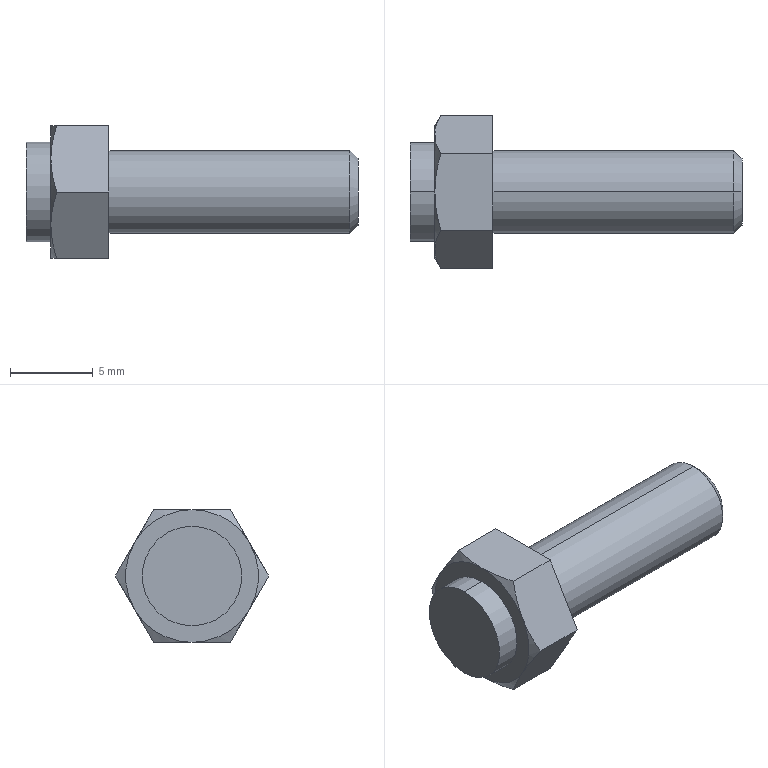Component | SolidWorks | USTH5-15-1_1-1 | 1 solid | 29 faces | box 20 x 9.24 x 8 mm | volume 510 mm3 | plane 17 | cone 8 | cylinder 4 | commonest cylinder face diameters 5 x2 6 x2
STEP:
#1=CARTESIAN_POINT('',(18.798,0.9252,2.854));
#2=VERTEX_POINT('',#1);
#3=CARTESIAN_POINT('',(18.798,0.9252,3.051));
#4=VERTEX_POINT('',#3);
#5=CARTESIAN_POINT('',(18.798,0.9252,2.953));
#6=DIRECTION('',(1.,0.,0.));
#7=DIRECTION('',(0.,0.,-1.));
#8=AXIS2_PLACEMENT_3D('',#5,#6,#7);
#9=CIRCLE('',#8,0.09843);
#10=EDGE_CURVE('',#2,#4,#9,.T.);
#11=ORIENTED_EDGE('',*,*,#10,.T.);
#12=CARTESIAN_POINT('',(19.37,0.9252,3.051));
#13=VERTEX_POINT('',#12);
#14=CARTESIAN_POINT('',(19.084,0.9252,3.051));
#15=DIRECTION('',(1.,0.,0.));
#16=VECTOR('',#15,39.37);
#17=LINE('',#14,#16);
#18=EDGE_CURVE('',#4,#13,#17,.T.);
#19=ORIENTED_EDGE('',*,*,#18,.T.);
#20=CARTESIAN_POINT('',(19.37,0.9252,2.854));
#21=VERTEX_POINT('',#20);
#22=CARTESIAN_POINT('',(19.37,0.9252,2.953));
#23=DIRECTION('',(-1.,0.,0.));
#24=DIRECTION('',(0.,0.,-1.));
#25=AXIS2_PLACEMENT_3D('',#22,#23,#24);
#26=CIRCLE('',#25,0.09843);
#27=EDGE_CURVE('',#13,#21,#26,.T.);
#28=ORIENTED_EDGE('',*,*,#27,.T.);
#29=CARTESIAN_POINT('',(19.084,0.9252,2.854));
#30=DIRECTION('',(1.,0.,0.));
#31=VECTOR('',#30,39.37);
#32=LINE('',#29,#31);
#33=EDGE_CURVE('',#2,#21,#32,.T.);
#34=ORIENTED_EDGE('',*,*,#33,.F.);
#35=EDGE_LOOP('',(#11,#19,#28,#34));
#36=FACE_OUTER_BOUND('',#35,.T.);
#37=CARTESIAN_POINT('',(19.084,0.9252,2.953));
#38=DIRECTION('',(1.,0.,0.));
#39=DIRECTION('',(0.,0.,-1.));
#40=AXIS2_PLACEMENT_3D('',#37,#38,#39);
#41=CYLINDRICAL_SURFACE('',#40,0.09843);
#42=ADVANCED_FACE('',(#36),#41,.T.);
#43=CARTESIAN_POINT('',(19.389,0.9252,3.032));
#44=VERTEX_POINT('',#43);
#45=CARTESIAN_POINT('',(19.389,0.9252,2.874));
#46=VERTEX_POINT('',#45);
#47=CARTESIAN_POINT('',(19.389,0.9252,2.953));
#48=DIRECTION('',(-1.,0.,0.));
#49=DIRECTION('',(0.,0.,1.));
#50=AXIS2_PLACEMENT_3D('',#47,#48,#49);
#51=CIRCLE('',#50,0.07911);
#52=EDGE_CURVE('',#44,#46,#51,.T.);
#53=ORIENTED_EDGE('',*,*,#52,.T.);
#54=CARTESIAN_POINT('',(19.37,0.9252,2.854));
#55=DIRECTION('',(-0.7071,0.,-0.7071));
#56=VECTOR('',#55,39.37);
#57=LINE('',#54,#56);
#58=EDGE_CURVE('',#46,#21,#57,.T.);
#59=ORIENTED_EDGE('',*,*,#58,.T.);
#60=ORIENTED_EDGE('',*,*,#27,.F.);
#61=CARTESIAN_POINT('',(19.37,0.9252,3.051));
#62=DIRECTION('',(-0.7071,0.,0.7071));
#63=VECTOR('',#62,39.37);
#64=LINE('',#61,#63);
#65=EDGE_CURVE('',#44,#13,#64,.T.);
#66=ORIENTED_EDGE('',*,*,#65,.F.);
#67=EDGE_LOOP('',(#53,#59,#60,#66));
#68=FACE_OUTER_BOUND('',#67,.T.);
#69=CARTESIAN_POINT('',(19.37,0.9252,2.953));
#70=DIRECTION('',(-1.,0.,0.));
#71=DIRECTION('',(0.,0.,1.));
#72=AXIS2_PLACEMENT_3D('',#69,#70,#71);
#73=CONICAL_SURFACE('',#72,0.09843,0.7854);
#74=ADVANCED_FACE('',(#68),#73,.T.);
#75=CARTESIAN_POINT('',(18.602,0.9252,2.835));
#76=VERTEX_POINT('',#75);
#77=CARTESIAN_POINT('',(18.602,0.9252,3.071));
#78=VERTEX_POINT('',#77);
#79=CARTESIAN_POINT('',(18.602,0.9252,2.953));
#80=DIRECTION('',(1.,0.,0.));
#81=DIRECTION('',(0.,0.,-1.));
#82=AXIS2_PLACEMENT_3D('',#79,#80,#81);
#83=CIRCLE('',#82,0.1181);
#84=EDGE_CURVE('',#76,#78,#83,.T.);
#85=ORIENTED_EDGE('',*,*,#84,.T.);
#86=CARTESIAN_POINT('',(18.661,0.9252,3.071));
#87=VERTEX_POINT('',#86);
#88=CARTESIAN_POINT('',(18.631,0.9252,3.071));
#89=DIRECTION('',(1.,0.,0.));
#90=VECTOR('',#89,39.37);
#91=LINE('',#88,#90);
#92=EDGE_CURVE('',#78,#87,#91,.T.);
#93=ORIENTED_EDGE('',*,*,#92,.T.);
#94=CARTESIAN_POINT('',(18.661,0.9252,2.835));
#95=VERTEX_POINT('',#94);
#96=CARTESIAN_POINT('',(18.661,0.9252,2.953));
#97=DIRECTION('',(1.,0.,0.));
#98=DIRECTION('',(0.,0.,-1.));
#99=AXIS2_PLACEMENT_3D('',#96,#97,#98);
#100=CIRCLE('',#99,0.1181);
#101=EDGE_CURVE('',#95,#87,#100,.T.);
#102=ORIENTED_EDGE('',*,*,#101,.F.);
#103=CARTESIAN_POINT('',(18.631,0.9252,2.835));
#104=DIRECTION('',(1.,0.,0.));
#105=VECTOR('',#104,39.37);
#106=LINE('',#103,#105);
#107=EDGE_CURVE('',#76,#95,#106,.T.);
#108=ORIENTED_EDGE('',*,*,#107,.F.);
#109=EDGE_LOOP('',(#85,#93,#102,#108));
#110=FACE_OUTER_BOUND('',#109,.T.);
#111=CARTESIAN_POINT('',(18.631,0.9252,2.953));
#112=DIRECTION('',(1.,0.,0.));
#113=DIRECTION('',(0.,0.,-1.));
#114=AXIS2_PLACEMENT_3D('',#111,#112,#113);
#115=CYLINDRICAL_SURFACE('',#114,0.1181);
#116=ADVANCED_FACE('',(#110),#115,.T.);
#117=ORIENTED_EDGE('',*,*,#18,.F.);
#118=CARTESIAN_POINT('',(18.798,0.9252,2.953));
#119=DIRECTION('',(1.,0.,0.));
#120=DIRECTION('',(0.,0.,-1.));
#121=AXIS2_PLACEMENT_3D('',#118,#119,#120);
#122=CIRCLE('',#121,0.09843);
#123=EDGE_CURVE('',#4,#2,#122,.T.);
#124=ORIENTED_EDGE('',*,*,#123,.T.);
#125=ORIENTED_EDGE('',*,*,#33,.T.);
#126=CARTESIAN_POINT('',(19.37,0.9252,2.953));
#127=DIRECTION('',(-1.,0.,0.));
#128=DIRECTION('',(0.,0.,-1.));
#129=AXIS2_PLACEMENT_3D('',#126,#127,#128);
#130=CIRCLE('',#129,0.09843);
#131=EDGE_CURVE('',#21,#13,#130,.T.);
#132=ORIENTED_EDGE('',*,*,#131,.T.);
#133=EDGE_LOOP('',(#117,#124,#125,#132));
#134=FACE_OUTER_BOUND('',#133,.T.);
#135=CARTESIAN_POINT('',(19.084,0.9252,2.953));
#136=DIRECTION('',(1.,0.,0.));
#137=DIRECTION('',(0.,0.,-1.));
#138=AXIS2_PLACEMENT_3D('',#135,#136,#137);
#139=CYLINDRICAL_SURFACE('',#138,0.09843);
#140=ADVANCED_FACE('',(#134),#139,.T.);
#141=ORIENTED_EDGE('',*,*,#10,.F.);
#142=ORIENTED_EDGE('',*,*,#123,.F.);
#143=EDGE_LOOP('',(#141,#142));
#144=FACE_BOUND('',#143,.T.);
#145=CARTESIAN_POINT('',(18.798,0.7434,2.953));
#146=VERTEX_POINT('',#145);
#147=CARTESIAN_POINT('',(18.798,0.8343,2.795));
#148=VERTEX_POINT('',#147);
#149=CARTESIAN_POINT('',(18.798,0.7434,2.953));
#150=DIRECTION('',(0.,0.5,-0.866));
#151=VECTOR('',#150,39.37);
#152=LINE('',#149,#151);
#153=EDGE_CURVE('',#146,#148,#152,.T.);
#154=ORIENTED_EDGE('',*,*,#153,.T.);
#155=CARTESIAN_POINT('',(18.798,1.016,2.795));
#156=VERTEX_POINT('',#155);
#157=CARTESIAN_POINT('',(18.798,1.069,2.795));
#158=DIRECTION('',(0.,1.,0.));
#159=VECTOR('',#158,39.37);
#160=LINE('',#157,#159);
#161=EDGE_CURVE('',#148,#156,#160,.T.);
#162=ORIENTED_EDGE('',*,*,#161,.T.);
#163=CARTESIAN_POINT('',(18.798,1.107,2.953));
#164=VERTEX_POINT('',#163);
#165=CARTESIAN_POINT('',(18.798,1.016,2.795));
#166=DIRECTION('',(0.,0.5,0.866));
#167=VECTOR('',#166,39.37);
#168=LINE('',#165,#167);
#169=EDGE_CURVE('',#156,#164,#168,.T.);
#170=ORIENTED_EDGE('',*,*,#169,.T.);
#171=CARTESIAN_POINT('',(18.798,1.016,3.11));
#172=VERTEX_POINT('',#171);
#173=CARTESIAN_POINT('',(18.798,1.107,2.953));
#174=DIRECTION('',(0.,-0.5,0.866));
#175=VECTOR('',#174,39.37);
#176=LINE('',#173,#175);
#177=EDGE_CURVE('',#164,#172,#176,.T.);
#178=ORIENTED_EDGE('',*,*,#177,.T.);
#179=CARTESIAN_POINT('',(18.798,0.8343,3.11));
#180=VERTEX_POINT('',#179);
#181=CARTESIAN_POINT('',(18.798,1.069,3.11));
#182=DIRECTION('',(0.,-1.,0.));
#183=VECTOR('',#182,39.37);
#184=LINE('',#181,#183);
#185=EDGE_CURVE('',#172,#180,#184,.T.);
#186=ORIENTED_EDGE('',*,*,#185,.T.);
#187=CARTESIAN_POINT('',(18.798,0.8343,3.11));
#188=DIRECTION('',(0.,-0.5,-0.866));
#189=VECTOR('',#188,39.37);
#190=LINE('',#187,#189);
#191=EDGE_CURVE('',#180,#146,#190,.T.);
#192=ORIENTED_EDGE('',*,*,#191,.T.);
#193=EDGE_LOOP('',(#154,#162,#170,#178,#186,#192));
#194=FACE_OUTER_BOUND('',#193,.T.);
#195=CARTESIAN_POINT('',(18.798,1.069,2.953));
#196=DIRECTION('',(1.,0.,0.));
#197=DIRECTION('',(0.,0.,-1.));
#198=AXIS2_PLACEMENT_3D('',#195,#196,#197);
#199=PLANE('',#198);
#200=ADVANCED_FACE('',(#144,#194),#199,.T.);
#201=ORIENTED_EDGE('',*,*,#58,.F.);
#202=CARTESIAN_POINT('',(19.389,0.9252,2.953));
#203=DIRECTION('',(-1.,0.,0.));
#204=DIRECTION('',(0.,0.,1.));
#205=AXIS2_PLACEMENT_3D('',#202,#203,#204);
#206=CIRCLE('',#205,0.07911);
#207=EDGE_CURVE('',#46,#44,#206,.T.);
#208=ORIENTED_EDGE('',*,*,#207,.T.);
#209=ORIENTED_EDGE('',*,*,#65,.T.);
#210=ORIENTED_EDGE('',*,*,#131,.F.);
#211=EDGE_LOOP('',(#201,#208,#209,#210));
#212=FACE_OUTER_BOUND('',#211,.T.);
#213=CARTESIAN_POINT('',(19.37,0.9252,2.953));
#214=DIRECTION('',(-1.,0.,0.));
#215=DIRECTION('',(0.,0.,1.));
#216=AXIS2_PLACEMENT_3D('',#213,#214,#215);
#217=CONICAL_SURFACE('',#216,0.09843,0.7854);
#218=ADVANCED_FACE('',(#212),#217,.T.);
#219=CARTESIAN_POINT('',(18.675,1.016,2.795));
#220=VERTEX_POINT('',#219);
#221=CARTESIAN_POINT('',(18.661,0.9252,2.795));
#222=VERTEX_POINT('',#221);
#223=CARTESIAN_POINT('',(18.675,1.016,2.795));
#224=CARTESIAN_POINT('',(18.666,0.9864,2.795));
#225=CARTESIAN_POINT('',(18.661,0.9562,2.795));
#226=CARTESIAN_POINT('',(18.661,0.9252,2.795));
#227=B_SPLINE_CURVE_WITH_KNOTS('',3,(#223,#224,#225,#226),.UNSPECIFIED.,.F.,.F.,(4,4),(0.,0.002337),.UNSPECIFIED.);
#228=EDGE_CURVE('',#220,#222,#227,.T.);
#229=ORIENTED_EDGE('',*,*,#228,.F.);
#230=CARTESIAN_POINT('',(18.798,1.016,2.795));
#231=DIRECTION('',(-1.,0.,0.));
#232=VECTOR('',#231,39.37);
#233=LINE('',#230,#232);
#234=EDGE_CURVE('',#156,#220,#233,.T.);
#235=ORIENTED_EDGE('',*,*,#234,.F.);
#236=ORIENTED_EDGE('',*,*,#161,.F.);
#237=CARTESIAN_POINT('',(18.675,0.8343,2.795));
#238=VERTEX_POINT('',#237);
#239=CARTESIAN_POINT('',(18.798,0.8343,2.795));
#240=DIRECTION('',(1.,0.,0.));
#241=VECTOR('',#240,39.37);
#242=LINE('',#239,#241);
#243=EDGE_CURVE('',#238,#148,#242,.T.);
#244=ORIENTED_EDGE('',*,*,#243,.F.);
#245=CARTESIAN_POINT('',(18.661,0.9252,2.795));
#246=CARTESIAN_POINT('',(18.661,0.8942,2.795));
#247=CARTESIAN_POINT('',(18.666,0.864,2.795));
#248=CARTESIAN_POINT('',(18.675,0.8343,2.795));
#249=B_SPLINE_CURVE_WITH_KNOTS('',3,(#245,#246,#247,#248),.UNSPECIFIED.,.F.,.F.,(4,4),(0.,0.002337),.UNSPECIFIED.);
#250=EDGE_CURVE('',#222,#238,#249,.T.);
#251=ORIENTED_EDGE('',*,*,#250,.F.);
#252=EDGE_LOOP('',(#229,#235,#236,#244,#251));
#253=FACE_OUTER_BOUND('',#252,.T.);
#254=CARTESIAN_POINT('',(18.798,1.016,2.795));
#255=DIRECTION('',(0.,0.,1.));
#256=DIRECTION('',(1.,0.,0.));
#257=AXIS2_PLACEMENT_3D('',#254,#255,#256);
#258=PLANE('',#257);
#259=ADVANCED_FACE('',(#253),#258,.F.);
#260=CARTESIAN_POINT('',(18.661,0.7888,2.874));
#261=VERTEX_POINT('',#260);
#262=CARTESIAN_POINT('',(18.675,0.8343,2.795));
#263=CARTESIAN_POINT('',(18.666,0.8194,2.821));
#264=CARTESIAN_POINT('',(18.661,0.8043,2.847));
#265=CARTESIAN_POINT('',(18.661,0.7888,2.874));
#266=B_SPLINE_CURVE_WITH_KNOTS('',3,(#262,#263,#264,#265),.UNSPECIFIED.,.F.,.F.,(4,4),(0.,0.002337),.UNSPECIFIED.);
#267=EDGE_CURVE('',#238,#261,#266,.T.);
#268=ORIENTED_EDGE('',*,*,#267,.F.);
#269=ORIENTED_EDGE('',*,*,#243,.T.);
#270=ORIENTED_EDGE('',*,*,#153,.F.);
#271=CARTESIAN_POINT('',(18.675,0.7434,2.953));
#272=VERTEX_POINT('',#271);
#273=CARTESIAN_POINT('',(18.798,0.7434,2.953));
#274=DIRECTION('',(1.,0.,0.));
#275=VECTOR('',#274,39.37);
#276=LINE('',#273,#275);
#277=EDGE_CURVE('',#272,#146,#276,.T.);
#278=ORIENTED_EDGE('',*,*,#277,.F.);
#279=CARTESIAN_POINT('',(18.661,0.7888,2.874));
#280=CARTESIAN_POINT('',(18.661,0.7733,2.901));
#281=CARTESIAN_POINT('',(18.666,0.7582,2.927));
#282=CARTESIAN_POINT('',(18.675,0.7434,2.953));
#283=B_SPLINE_CURVE_WITH_KNOTS('',3,(#279,#280,#281,#282),.UNSPECIFIED.,.F.,.F.,(4,4),(0.,0.002337),.UNSPECIFIED.);
#284=EDGE_CURVE('',#261,#272,#283,.T.);
#285=ORIENTED_EDGE('',*,*,#284,.F.);
#286=EDGE_LOOP('',(#268,#269,#270,#278,#285));
#287=FACE_OUTER_BOUND('',#286,.T.);
#288=CARTESIAN_POINT('',(18.798,0.8343,2.795));
#289=DIRECTION('',(0.,0.866,0.5));
#290=DIRECTION('',(0.,-0.5,0.866));
#291=AXIS2_PLACEMENT_3D('',#288,#289,#290);
#292=PLANE('',#291);
#293=ADVANCED_FACE('',(#287),#292,.F.);
#294=ORIENTED_EDGE('',*,*,#277,.T.);
#295=ORIENTED_EDGE('',*,*,#191,.F.);
#296=CARTESIAN_POINT('',(18.675,0.8343,3.11));
#297=VERTEX_POINT('',#296);
#298=CARTESIAN_POINT('',(18.798,0.8343,3.11));
#299=DIRECTION('',(1.,0.,0.));
#300=VECTOR('',#299,39.37);
#301=LINE('',#298,#300);
#302=EDGE_CURVE('',#297,#180,#301,.T.);
#303=ORIENTED_EDGE('',*,*,#302,.F.);
#304=CARTESIAN_POINT('',(18.661,0.7888,3.031));
#305=VERTEX_POINT('',#304);
#306=CARTESIAN_POINT('',(18.661,0.7888,3.031));
#307=CARTESIAN_POINT('',(18.661,0.8043,3.058));
#308=CARTESIAN_POINT('',(18.666,0.8194,3.085));
#309=CARTESIAN_POINT('',(18.675,0.8343,3.11));
#310=B_SPLINE_CURVE_WITH_KNOTS('',3,(#306,#307,#308,#309),.UNSPECIFIED.,.F.,.F.,(4,4),(0.,0.002337),.UNSPECIFIED.);
#311=EDGE_CURVE('',#305,#297,#310,.T.);
#312=ORIENTED_EDGE('',*,*,#311,.F.);
#313=CARTESIAN_POINT('',(18.675,0.7434,2.953));
#314=CARTESIAN_POINT('',(18.666,0.7582,2.978));
#315=CARTESIAN_POINT('',(18.661,0.7733,3.005));
#316=CARTESIAN_POINT('',(18.661,0.7888,3.031));
#317=B_SPLINE_CURVE_WITH_KNOTS('',3,(#313,#314,#315,#316),.UNSPECIFIED.,.F.,.F.,(4,4),(0.,0.002337),.UNSPECIFIED.);
#318=EDGE_CURVE('',#272,#305,#317,.T.);
#319=ORIENTED_EDGE('',*,*,#318,.F.);
#320=EDGE_LOOP('',(#294,#295,#303,#312,#319));
#321=FACE_OUTER_BOUND('',#320,.T.);
#322=CARTESIAN_POINT('',(18.798,0.7434,2.953));
#323=DIRECTION('',(0.,0.866,-0.5));
#324=DIRECTION('',(0.,0.5,0.866));
#325=AXIS2_PLACEMENT_3D('',#322,#323,#324);
#326=PLANE('',#325);
#327=ADVANCED_FACE('',(#321),#326,.F.);
#328=ORIENTED_EDGE('',*,*,#302,.T.);
#329=ORIENTED_EDGE('',*,*,#185,.F.);
#330=CARTESIAN_POINT('',(18.675,1.016,3.11));
#331=VERTEX_POINT('',#330);
#332=CARTESIAN_POINT('',(18.798,1.016,3.11));
#333=DIRECTION('',(1.,0.,0.));
#334=VECTOR('',#333,39.37);
#335=LINE('',#332,#334);
#336=EDGE_CURVE('',#331,#172,#335,.T.);
#337=ORIENTED_EDGE('',*,*,#336,.F.);
#338=CARTESIAN_POINT('',(18.661,0.9252,3.11));
#339=VERTEX_POINT('',#338);
#340=CARTESIAN_POINT('',(18.661,0.9252,3.11));
#341=CARTESIAN_POINT('',(18.661,0.9562,3.11));
#342=CARTESIAN_POINT('',(18.666,0.9864,3.11));
#343=CARTESIAN_POINT('',(18.675,1.016,3.11));
#344=B_SPLINE_CURVE_WITH_KNOTS('',3,(#340,#341,#342,#343),.UNSPECIFIED.,.F.,.F.,(4,4),(0.,0.002337),.UNSPECIFIED.);
#345=EDGE_CURVE('',#339,#331,#344,.T.);
#346=ORIENTED_EDGE('',*,*,#345,.F.);
#347=CARTESIAN_POINT('',(18.675,0.8343,3.11));
#348=CARTESIAN_POINT('',(18.666,0.864,3.11));
#349=CARTESIAN_POINT('',(18.661,0.8942,3.11));
#350=CARTESIAN_POINT('',(18.661,0.9252,3.11));
#351=B_SPLINE_CURVE_WITH_KNOTS('',3,(#347,#348,#349,#350),.UNSPECIFIED.,.F.,.F.,(4,4),(0.,0.002337),.UNSPECIFIED.);
#352=EDGE_CURVE('',#297,#339,#351,.T.);
#353=ORIENTED_EDGE('',*,*,#352,.F.);
#354=EDGE_LOOP('',(#328,#329,#337,#346,#353));
#355=FACE_OUTER_BOUND('',#354,.T.);
#356=CARTESIAN_POINT('',(18.798,0.8343,3.11));
#357=DIRECTION('',(0.,0.,-1.));
#358=DIRECTION('',(-1.,0.,0.));
#359=AXIS2_PLACEMENT_3D('',#356,#357,#358);
#360=PLANE('',#359);
#361=ADVANCED_FACE('',(#355),#360,.F.);
#362=ORIENTED_EDGE('',*,*,#336,.T.);
#363=ORIENTED_EDGE('',*,*,#177,.F.);
#364=CARTESIAN_POINT('',(18.675,1.107,2.953));
#365=VERTEX_POINT('',#364);
#366=CARTESIAN_POINT('',(18.798,1.107,2.953));
#367=DIRECTION('',(1.,0.,0.));
#368=VECTOR('',#367,39.37);
#369=LINE('',#366,#368);
#370=EDGE_CURVE('',#365,#164,#369,.T.);
#371=ORIENTED_EDGE('',*,*,#370,.F.);
#372=CARTESIAN_POINT('',(18.661,1.062,3.031));
#373=VERTEX_POINT('',#372);
#374=CARTESIAN_POINT('',(18.661,1.062,3.031));
#375=CARTESIAN_POINT('',(18.661,1.077,3.005));
#376=CARTESIAN_POINT('',(18.666,1.092,2.978));
#377=CARTESIAN_POINT('',(18.675,1.107,2.953));
#378=B_SPLINE_CURVE_WITH_KNOTS('',3,(#374,#375,#376,#377),.UNSPECIFIED.,.F.,.F.,(4,4),(0.,0.002337),.UNSPECIFIED.);
#379=EDGE_CURVE('',#373,#365,#378,.T.);
#380=ORIENTED_EDGE('',*,*,#379,.F.);
#381=CARTESIAN_POINT('',(18.675,1.016,3.11));
#382=CARTESIAN_POINT('',(18.666,1.031,3.085));
#383=CARTESIAN_POINT('',(18.661,1.046,3.058));
#384=CARTESIAN_POINT('',(18.661,1.062,3.031));
#385=B_SPLINE_CURVE_WITH_KNOTS('',3,(#381,#382,#383,#384),.UNSPECIFIED.,.F.,.F.,(4,4),(0.,0.002337),.UNSPECIFIED.);
#386=EDGE_CURVE('',#331,#373,#385,.T.);
#387=ORIENTED_EDGE('',*,*,#386,.F.);
#388=EDGE_LOOP('',(#362,#363,#371,#380,#387));
#389=FACE_OUTER_BOUND('',#388,.T.);
#390=CARTESIAN_POINT('',(18.798,1.016,3.11));
#391=DIRECTION('',(0.,-0.866,-0.5));
#392=DIRECTION('',(0.,0.5,-0.866));
#393=AXIS2_PLACEMENT_3D('',#390,#391,#392);
#394=PLANE('',#393);
#395=ADVANCED_FACE('',(#389),#394,.F.);
#396=CARTESIAN_POINT('',(18.661,1.062,2.874));
#397=VERTEX_POINT('',#396);
#398=CARTESIAN_POINT('',(18.675,1.107,2.953));
#399=CARTESIAN_POINT('',(18.666,1.092,2.927));
#400=CARTESIAN_POINT('',(18.661,1.077,2.901));
#401=CARTESIAN_POINT('',(18.661,1.062,2.874));
#402=B_SPLINE_CURVE_WITH_KNOTS('',3,(#398,#399,#400,#401),.UNSPECIFIED.,.F.,.F.,(4,4),(0.,0.002337),.UNSPECIFIED.);
#403=EDGE_CURVE('',#365,#397,#402,.T.);
#404=ORIENTED_EDGE('',*,*,#403,.F.);
#405=ORIENTED_EDGE('',*,*,#370,.T.);
#406=ORIENTED_EDGE('',*,*,#169,.F.);
#407=ORIENTED_EDGE('',*,*,#234,.T.);
#408=CARTESIAN_POINT('',(18.661,1.062,2.874));
#409=CARTESIAN_POINT('',(18.661,1.046,2.847));
#410=CARTESIAN_POINT('',(18.666,1.031,2.821));
#411=CARTESIAN_POINT('',(18.675,1.016,2.795));
#412=B_SPLINE_CURVE_WITH_KNOTS('',3,(#408,#409,#410,#411),.UNSPECIFIED.,.F.,.F.,(4,4),(0.,0.002337),.UNSPECIFIED.);
#413=EDGE_CURVE('',#397,#220,#412,.T.);
#414=ORIENTED_EDGE('',*,*,#413,.F.);
#415=EDGE_LOOP('',(#404,#405,#406,#407,#414));
#416=FACE_OUTER_BOUND('',#415,.T.);
#417=CARTESIAN_POINT('',(18.798,1.107,2.953));
#418=DIRECTION('',(0.,-0.866,0.5));
#419=DIRECTION('',(0.,-0.5,-0.866));
#420=AXIS2_PLACEMENT_3D('',#417,#418,#419);
#421=PLANE('',#420);
#422=ADVANCED_FACE('',(#416),#421,.F.);
#423=ORIENTED_EDGE('',*,*,#52,.F.);
#424=ORIENTED_EDGE('',*,*,#207,.F.);
#425=EDGE_LOOP('',(#423,#424));
#426=FACE_OUTER_BOUND('',#425,.T.);
#427=CARTESIAN_POINT('',(19.389,0.957,2.898));
#428=VERTEX_POINT('',#427);
#429=CARTESIAN_POINT('',(19.389,0.8934,2.898));
#430=VERTEX_POINT('',#429);
#431=CARTESIAN_POINT('',(19.389,0.8934,2.898));
#432=DIRECTION('',(0.,-1.,0.));
#433=VECTOR('',#432,39.37);
#434=LINE('',#431,#433);
#435=EDGE_CURVE('',#428,#430,#434,.T.);
#436=ORIENTED_EDGE('',*,*,#435,.T.);
#437=CARTESIAN_POINT('',(19.389,0.8616,2.953));
#438=VERTEX_POINT('',#437);
#439=CARTESIAN_POINT('',(19.389,0.8934,2.898));
#440=DIRECTION('',(0.,-0.5,0.866));
#441=VECTOR('',#440,39.37);
#442=LINE('',#439,#441);
#443=EDGE_CURVE('',#430,#438,#442,.T.);
#444=ORIENTED_EDGE('',*,*,#443,.T.);
#445=CARTESIAN_POINT('',(19.389,0.8934,3.008));
#446=VERTEX_POINT('',#445);
#447=CARTESIAN_POINT('',(19.389,0.8934,3.008));
#448=DIRECTION('',(0.,0.5,0.866));
#449=VECTOR('',#448,39.37);
#450=LINE('',#447,#449);
#451=EDGE_CURVE('',#438,#446,#450,.T.);
#452=ORIENTED_EDGE('',*,*,#451,.T.);
#453=CARTESIAN_POINT('',(19.389,0.957,3.008));
#454=VERTEX_POINT('',#453);
#455=CARTESIAN_POINT('',(19.389,0.957,3.008));
#456=DIRECTION('',(0.,1.,0.));
#457=VECTOR('',#456,39.37);
#458=LINE('',#455,#457);
#459=EDGE_CURVE('',#446,#454,#458,.T.);
#460=ORIENTED_EDGE('',*,*,#459,.T.);
#461=CARTESIAN_POINT('',(19.389,0.9888,2.953));
#462=VERTEX_POINT('',#461);
#463=CARTESIAN_POINT('',(19.389,0.9888,2.953));
#464=DIRECTION('',(0.,0.5,-0.866));
#465=VECTOR('',#464,39.37);
#466=LINE('',#463,#465);
#467=EDGE_CURVE('',#454,#462,#466,.T.);
#468=ORIENTED_EDGE('',*,*,#467,.T.);
#469=CARTESIAN_POINT('',(19.389,0.957,2.898));
#470=DIRECTION('',(0.,-0.5,-0.866));
#471=VECTOR('',#470,39.37);
#472=LINE('',#469,#471);
#473=EDGE_CURVE('',#462,#428,#472,.T.);
#474=ORIENTED_EDGE('',*,*,#473,.T.);
#475=EDGE_LOOP('',(#436,#444,#452,#460,#468,#474));
#476=FACE_BOUND('',#475,.T.);
#477=CARTESIAN_POINT('',(19.389,0.9648,2.953));
#478=DIRECTION('',(1.,0.,0.));
#479=DIRECTION('',(0.,0.,-1.));
#480=AXIS2_PLACEMENT_3D('',#477,#478,#479);
#481=PLANE('',#480);
#482=ADVANCED_FACE('',(#426,#476),#481,.T.);
#483=CARTESIAN_POINT('',(18.661,0.9252,2.953));
#484=DIRECTION('',(1.,0.,0.));
#485=DIRECTION('',(0.,0.,-1.));
#486=AXIS2_PLACEMENT_3D('',#483,#484,#485);
#487=CIRCLE('',#486,0.1575);
#488=EDGE_CURVE('',#261,#222,#487,.T.);
#489=ORIENTED_EDGE('',*,*,#488,.T.);
#490=ORIENTED_EDGE('',*,*,#250,.T.);
#491=ORIENTED_EDGE('',*,*,#267,.T.);
#492=EDGE_LOOP('',(#489,#490,#491));
#493=FACE_OUTER_BOUND('',#492,.T.);
#494=CARTESIAN_POINT('',(18.675,0.9252,2.953));
#495=DIRECTION('',(1.,0.,0.));
#496=DIRECTION('',(0.,0.,-1.));
#497=AXIS2_PLACEMENT_3D('',#494,#495,#496);
#498=CONICAL_SURFACE('',#497,0.182,1.047);
#499=ADVANCED_FACE('',(#493),#498,.T.);
#500=CARTESIAN_POINT('',(18.661,0.9252,2.953));
#501=DIRECTION('',(1.,0.,0.));
#502=DIRECTION('',(0.,0.,-1.));
#503=AXIS2_PLACEMENT_3D('',#500,#501,#502);
#504=CIRCLE('',#503,0.1575);
#505=EDGE_CURVE('',#222,#397,#504,.T.);
#506=ORIENTED_EDGE('',*,*,#505,.T.);
#507=ORIENTED_EDGE('',*,*,#413,.T.);
#508=ORIENTED_EDGE('',*,*,#228,.T.);
#509=EDGE_LOOP('',(#506,#507,#508));
#510=FACE_OUTER_BOUND('',#509,.T.);
#511=CARTESIAN_POINT('',(18.675,0.9252,2.953));
#512=DIRECTION('',(1.,0.,0.));
#513=DIRECTION('',(0.,0.,-1.));
#514=AXIS2_PLACEMENT_3D('',#511,#512,#513);
#515=CONICAL_SURFACE('',#514,0.182,1.047);
#516=ADVANCED_FACE('',(#510),#515,.T.);
#517=CARTESIAN_POINT('',(18.661,0.9252,2.953));
#518=DIRECTION('',(1.,0.,0.));
#519=DIRECTION('',(0.,0.,-1.));
#520=AXIS2_PLACEMENT_3D('',#517,#518,#519);
#521=CIRCLE('',#520,0.1575);
#522=EDGE_CURVE('',#305,#261,#521,.T.);
#523=ORIENTED_EDGE('',*,*,#522,.T.);
#524=ORIENTED_EDGE('',*,*,#284,.T.);
#525=ORIENTED_EDGE('',*,*,#318,.T.);
#526=EDGE_LOOP('',(#523,#524,#525));
#527=FACE_OUTER_BOUND('',#526,.T.);
#528=CARTESIAN_POINT('',(18.675,0.9252,2.953));
#529=DIRECTION('',(1.,0.,0.));
#530=DIRECTION('',(0.,0.,-1.));
#531=AXIS2_PLACEMENT_3D('',#528,#529,#530);
#532=CONICAL_SURFACE('',#531,0.182,1.047);
#533=ADVANCED_FACE('',(#527),#532,.T.);
#534=ORIENTED_EDGE('',*,*,#352,.T.);
#535=CARTESIAN_POINT('',(18.661,0.9252,2.953));
#536=DIRECTION('',(1.,0.,0.));
#537=DIRECTION('',(0.,0.,-1.));
#538=AXIS2_PLACEMENT_3D('',#535,#536,#537);
#539=CIRCLE('',#538,0.1575);
#540=EDGE_CURVE('',#339,#305,#539,.T.);
#541=ORIENTED_EDGE('',*,*,#540,.T.);
#542=ORIENTED_EDGE('',*,*,#311,.T.);
#543=EDGE_LOOP('',(#534,#541,#542));
#544=FACE_OUTER_BOUND('',#543,.T.);
#545=CARTESIAN_POINT('',(18.675,0.9252,2.953));
#546=DIRECTION('',(1.,0.,0.));
#547=DIRECTION('',(0.,0.,-1.));
#548=AXIS2_PLACEMENT_3D('',#545,#546,#547);
#549=CONICAL_SURFACE('',#548,0.182,1.047);
#550=ADVANCED_FACE('',(#544),#549,.T.);
#551=ORIENTED_EDGE('',*,*,#386,.T.);
#552=CARTESIAN_POINT('',(18.661,0.9252,2.953));
#553=DIRECTION('',(1.,0.,0.));
#554=DIRECTION('',(0.,0.,-1.));
#555=AXIS2_PLACEMENT_3D('',#552,#553,#554);
#556=CIRCLE('',#555,0.1575);
#557=EDGE_CURVE('',#373,#339,#556,.T.);
#558=ORIENTED_EDGE('',*,*,#557,.T.);
#559=ORIENTED_EDGE('',*,*,#345,.T.);
#560=EDGE_LOOP('',(#551,#558,#559));
#561=FACE_OUTER_BOUND('',#560,.T.);
#562=CARTESIAN_POINT('',(18.675,0.9252,2.953));
#563=DIRECTION('',(1.,0.,0.));
#564=DIRECTION('',(0.,0.,-1.));
#565=AXIS2_PLACEMENT_3D('',#562,#563,#564);
#566=CONICAL_SURFACE('',#565,0.182,1.047);
#567=ADVANCED_FACE('',(#561),#566,.T.);
#568=CARTESIAN_POINT('',(18.661,0.9252,2.953));
#569=DIRECTION('',(1.,0.,0.));
#570=DIRECTION('',(0.,0.,-1.));
#571=AXIS2_PLACEMENT_3D('',#568,#569,#570);
#572=CIRCLE('',#571,0.1575);
#573=EDGE_CURVE('',#397,#373,#572,.T.);
#574=ORIENTED_EDGE('',*,*,#573,.T.);
#575=ORIENTED_EDGE('',*,*,#379,.T.);
#576=ORIENTED_EDGE('',*,*,#403,.T.);
#577=EDGE_LOOP('',(#574,#575,#576));
#578=FACE_OUTER_BOUND('',#577,.T.);
#579=CARTESIAN_POINT('',(18.675,0.9252,2.953));
#580=DIRECTION('',(1.,0.,0.));
#581=DIRECTION('',(0.,0.,-1.));
#582=AXIS2_PLACEMENT_3D('',#579,#580,#581);
#583=CONICAL_SURFACE('',#582,0.182,1.047);
#584=ADVANCED_FACE('',(#578),#583,.T.);
#585=CARTESIAN_POINT('',(19.279,0.8616,2.953));
#586=VERTEX_POINT('',#585);
#587=CARTESIAN_POINT('',(19.389,0.8616,2.953));
#588=DIRECTION('',(-1.,0.,0.));
#589=VECTOR('',#588,39.37);
#590=LINE('',#587,#589);
#591=EDGE_CURVE('',#438,#586,#590,.T.);
#592=ORIENTED_EDGE('',*,*,#591,.F.);
#593=ORIENTED_EDGE('',*,*,#443,.F.);
#594=CARTESIAN_POINT('',(19.279,0.8934,2.898));
#595=VERTEX_POINT('',#594);
#596=CARTESIAN_POINT('',(19.389,0.8934,2.898));
#597=DIRECTION('',(1.,0.,0.));
#598=VECTOR('',#597,39.37);
#599=LINE('',#596,#598);
#600=EDGE_CURVE('',#595,#430,#599,.T.);
#601=ORIENTED_EDGE('',*,*,#600,.F.);
#602=CARTESIAN_POINT('',(19.279,0.8616,2.953));
#603=DIRECTION('',(0.,0.5,-0.866));
#604=VECTOR('',#603,39.37);
#605=LINE('',#602,#604);
#606=EDGE_CURVE('',#586,#595,#605,.T.);
#607=ORIENTED_EDGE('',*,*,#606,.F.);
#608=EDGE_LOOP('',(#592,#593,#601,#607));
#609=FACE_OUTER_BOUND('',#608,.T.);
#610=CARTESIAN_POINT('',(19.389,0.8616,2.953));
#611=DIRECTION('',(0.,-0.866,-0.5));
#612=DIRECTION('',(0.,0.5,-0.866));
#613=AXIS2_PLACEMENT_3D('',#610,#611,#612);
#614=PLANE('',#613);
#615=ADVANCED_FACE('',(#609),#614,.F.);
#616=ORIENTED_EDGE('',*,*,#540,.F.);
#617=ORIENTED_EDGE('',*,*,#557,.F.);
#618=ORIENTED_EDGE('',*,*,#573,.F.);
#619=ORIENTED_EDGE('',*,*,#505,.F.);
#620=ORIENTED_EDGE('',*,*,#488,.F.);
#621=ORIENTED_EDGE('',*,*,#522,.F.);
#622=EDGE_LOOP('',(#616,#617,#618,#619,#620,#621));
#623=FACE_OUTER_BOUND('',#622,.T.);
#624=ORIENTED_EDGE('',*,*,#101,.T.);
#625=CARTESIAN_POINT('',(18.661,0.9252,2.953));
#626=DIRECTION('',(1.,0.,0.));
#627=DIRECTION('',(0.,0.,-1.));
#628=AXIS2_PLACEMENT_3D('',#625,#626,#627);
#629=CIRCLE('',#628,0.1181);
#630=EDGE_CURVE('',#87,#95,#629,.T.);
#631=ORIENTED_EDGE('',*,*,#630,.T.);
#632=EDGE_LOOP('',(#624,#631));
#633=FACE_BOUND('',#632,.T.);
#634=CARTESIAN_POINT('',(18.661,1.063,2.953));
#635=DIRECTION('',(-1.,0.,0.));
#636=DIRECTION('',(0.,0.,1.));
#637=AXIS2_PLACEMENT_3D('',#634,#635,#636);
#638=PLANE('',#637);
#639=ADVANCED_FACE('',(#623,#633),#638,.T.);
#640=CARTESIAN_POINT('',(19.279,0.9888,2.953));
#641=VERTEX_POINT('',#640);
#642=CARTESIAN_POINT('',(19.279,0.957,3.008));
#643=VERTEX_POINT('',#642);
#644=CARTESIAN_POINT('',(19.279,0.9888,2.953));
#645=DIRECTION('',(0.,-0.5,0.866));
#646=VECTOR('',#645,39.37);
#647=LINE('',#644,#646);
#648=EDGE_CURVE('',#641,#643,#647,.T.);
#649=ORIENTED_EDGE('',*,*,#648,.T.);
#650=CARTESIAN_POINT('',(19.279,0.8934,3.008));
#651=VERTEX_POINT('',#650);
#652=CARTESIAN_POINT('',(19.279,0.957,3.008));
#653=DIRECTION('',(0.,-1.,0.));
#654=VECTOR('',#653,39.37);
#655=LINE('',#652,#654);
#656=EDGE_CURVE('',#643,#651,#655,.T.);
#657=ORIENTED_EDGE('',*,*,#656,.T.);
#658=CARTESIAN_POINT('',(19.279,0.8934,3.008));
#659=DIRECTION('',(0.,-0.5,-0.866));
#660=VECTOR('',#659,39.37);
#661=LINE('',#658,#660);
#662=EDGE_CURVE('',#651,#586,#661,.T.);
#663=ORIENTED_EDGE('',*,*,#662,.T.);
#664=ORIENTED_EDGE('',*,*,#606,.T.);
#665=CARTESIAN_POINT('',(19.279,0.957,2.898));
#666=VERTEX_POINT('',#665);
#667=CARTESIAN_POINT('',(19.279,0.9252,2.898));
#668=DIRECTION('',(0.,1.,0.));
#669=VECTOR('',#668,39.37);
#670=LINE('',#667,#669);
#671=EDGE_CURVE('',#595,#666,#670,.T.);
#672=ORIENTED_EDGE('',*,*,#671,.T.);
#673=CARTESIAN_POINT('',(19.279,0.957,2.898));
#674=DIRECTION('',(0.,0.5,0.866));
#675=VECTOR('',#674,39.37);
#676=LINE('',#673,#675);
#677=EDGE_CURVE('',#666,#641,#676,.T.);
#678=ORIENTED_EDGE('',*,*,#677,.T.);
#679=EDGE_LOOP('',(#649,#657,#663,#664,#672,#678));
#680=FACE_OUTER_BOUND('',#679,.T.);
#681=CARTESIAN_POINT('',(19.279,0.9252,2.953));
#682=DIRECTION('',(1.,0.,0.));
#683=DIRECTION('',(0.,0.,-1.));
#684=AXIS2_PLACEMENT_3D('',#681,#682,#683);
#685=PLANE('',#684);
#686=ADVANCED_FACE('',(#680),#685,.T.);
#687=CARTESIAN_POINT('',(19.389,0.8934,3.008));
#688=DIRECTION('',(-1.,0.,0.));
#689=VECTOR('',#688,39.37);
#690=LINE('',#687,#689);
#691=EDGE_CURVE('',#446,#651,#690,.T.);
#692=ORIENTED_EDGE('',*,*,#691,.F.);
#693=ORIENTED_EDGE('',*,*,#451,.F.);
#694=ORIENTED_EDGE('',*,*,#591,.T.);
#695=ORIENTED_EDGE('',*,*,#662,.F.);
#696=EDGE_LOOP('',(#692,#693,#694,#695));
#697=FACE_OUTER_BOUND('',#696,.T.);
#698=CARTESIAN_POINT('',(19.389,0.8934,3.008));
#699=DIRECTION('',(0.,-0.866,0.5));
#700=DIRECTION('',(0.,-0.5,-0.866));
#701=AXIS2_PLACEMENT_3D('',#698,#699,#700);
#702=PLANE('',#701);
#703=ADVANCED_FACE('',(#697),#702,.F.);
#704=ORIENTED_EDGE('',*,*,#600,.T.);
#705=ORIENTED_EDGE('',*,*,#435,.F.);
#706=CARTESIAN_POINT('',(19.389,0.957,2.898));
#707=DIRECTION('',(1.,0.,0.));
#708=VECTOR('',#707,39.37);
#709=LINE('',#706,#708);
#710=EDGE_CURVE('',#666,#428,#709,.T.);
#711=ORIENTED_EDGE('',*,*,#710,.F.);
#712=ORIENTED_EDGE('',*,*,#671,.F.);
#713=EDGE_LOOP('',(#704,#705,#711,#712));
#714=FACE_OUTER_BOUND('',#713,.T.);
#715=CARTESIAN_POINT('',(19.389,0.8934,2.898));
#716=DIRECTION('',(0.,0.,-1.));
#717=DIRECTION('',(-1.,0.,0.));
#718=AXIS2_PLACEMENT_3D('',#715,#716,#717);
#719=PLANE('',#718);
#720=ADVANCED_FACE('',(#714),#719,.F.);
#721=ORIENTED_EDGE('',*,*,#92,.F.);
#722=CARTESIAN_POINT('',(18.602,0.9252,2.953));
#723=DIRECTION('',(1.,0.,0.));
#724=DIRECTION('',(0.,0.,-1.));
#725=AXIS2_PLACEMENT_3D('',#722,#723,#724);
#726=CIRCLE('',#725,0.1181);
#727=EDGE_CURVE('',#78,#76,#726,.T.);
#728=ORIENTED_EDGE('',*,*,#727,.T.);
#729=ORIENTED_EDGE('',*,*,#107,.T.);
#730=ORIENTED_EDGE('',*,*,#630,.F.);
#731=EDGE_LOOP('',(#721,#728,#729,#730));
#732=FACE_OUTER_BOUND('',#731,.T.);
#733=CARTESIAN_POINT('',(18.631,0.9252,2.953));
#734=DIRECTION('',(1.,0.,0.));
#735=DIRECTION('',(0.,0.,-1.));
#736=AXIS2_PLACEMENT_3D('',#733,#734,#735);
#737=CYLINDRICAL_SURFACE('',#736,0.1181);
#738=ADVANCED_FACE('',(#732),#737,.T.);
#739=CARTESIAN_POINT('',(19.389,0.957,3.008));
#740=DIRECTION('',(-1.,0.,0.));
#741=VECTOR('',#740,39.37);
#742=LINE('',#739,#741);
#743=EDGE_CURVE('',#454,#643,#742,.T.);
#744=ORIENTED_EDGE('',*,*,#743,.F.);
#745=ORIENTED_EDGE('',*,*,#459,.F.);
#746=ORIENTED_EDGE('',*,*,#691,.T.);
#747=ORIENTED_EDGE('',*,*,#656,.F.);
#748=EDGE_LOOP('',(#744,#745,#746,#747));
#749=FACE_OUTER_BOUND('',#748,.T.);
#750=CARTESIAN_POINT('',(19.389,0.957,3.008));
#751=DIRECTION('',(0.,0.,1.));
#752=DIRECTION('',(1.,0.,0.));
#753=AXIS2_PLACEMENT_3D('',#750,#751,#752);
#754=PLANE('',#753);
#755=ADVANCED_FACE('',(#749),#754,.F.);
#756=ORIENTED_EDGE('',*,*,#710,.T.);
#757=ORIENTED_EDGE('',*,*,#473,.F.);
#758=CARTESIAN_POINT('',(19.389,0.9888,2.953));
#759=DIRECTION('',(1.,0.,0.));
#760=VECTOR('',#759,39.37);
#761=LINE('',#758,#760);
#762=EDGE_CURVE('',#641,#462,#761,.T.);
#763=ORIENTED_EDGE('',*,*,#762,.F.);
#764=ORIENTED_EDGE('',*,*,#677,.F.);
#765=EDGE_LOOP('',(#756,#757,#763,#764));
#766=FACE_OUTER_BOUND('',#765,.T.);
#767=CARTESIAN_POINT('',(19.389,0.957,2.898));
#768=DIRECTION('',(0.,0.866,-0.5));
#769=DIRECTION('',(0.,0.5,0.866));
#770=AXIS2_PLACEMENT_3D('',#767,#768,#769);
#771=PLANE('',#770);
#772=ADVANCED_FACE('',(#766),#771,.F.);
#773=ORIENTED_EDGE('',*,*,#84,.F.);
#774=ORIENTED_EDGE('',*,*,#727,.F.);
#775=EDGE_LOOP('',(#773,#774));
#776=FACE_OUTER_BOUND('',#775,.T.);
#777=CARTESIAN_POINT('',(18.602,0.9843,2.953));
#778=DIRECTION('',(-1.,0.,0.));
#779=DIRECTION('',(0.,0.,1.));
#780=AXIS2_PLACEMENT_3D('',#777,#778,#779);
#781=PLANE('',#780);
#782=ADVANCED_FACE('',(#776),#781,.T.);
#783=ORIENTED_EDGE('',*,*,#762,.T.);
#784=ORIENTED_EDGE('',*,*,#467,.F.);
#785=ORIENTED_EDGE('',*,*,#743,.T.);
#786=ORIENTED_EDGE('',*,*,#648,.F.);
#787=EDGE_LOOP('',(#783,#784,#785,#786));
#788=FACE_OUTER_BOUND('',#787,.T.);
#789=CARTESIAN_POINT('',(19.389,0.9888,2.953));
#790=DIRECTION('',(0.,0.866,0.5));
#791=DIRECTION('',(0.,-0.5,0.866));
#792=AXIS2_PLACEMENT_3D('',#789,#790,#791);
#793=PLANE('',#792);
#794=ADVANCED_FACE('',(#788),#793,.F.);
#795=CLOSED_SHELL('',(#42,#74,#116,#140,#200,#218,#259,#293,#327,#361,#395,#422,#482,#499,#516,#533,#550,#567,#584,#615,#639,#686,#703,#720,#738,#755,#772,#782,#794));
#796=MANIFOLD_SOLID_BREP('',#795);
#797=CARTESIAN_POINT('',(0.,0.,0.));
#798=DIRECTION('',(0.,0.,1.));
#799=DIRECTION('',(1.,0.,0.));
#800=AXIS2_PLACEMENT_3D('',#797,#798,#799);
#801=(LENGTH_UNIT()NAMED_UNIT(*)SI_UNIT($,.METRE.));
#802=LENGTH_MEASURE_WITH_UNIT(LENGTH_MEASURE(0.0254),#801);
#803=DIMENSIONAL_EXPONENTS(1.,0.,0.,0.,0.,0.,0.);
#804=(CONVERSION_BASED_UNIT('',#802)LENGTH_UNIT()NAMED_UNIT(#803));
#805=UNCERTAINTY_MEASURE_WITH_UNIT(LENGTH_MEASURE(0.00001),#804,'','');
#806=(NAMED_UNIT(*)PLANE_ANGLE_UNIT()SI_UNIT($,.RADIAN.));
#807=(NAMED_UNIT(*)SI_UNIT($,.STERADIAN.)SOLID_ANGLE_UNIT());
#808=(GEOMETRIC_REPRESENTATION_CONTEXT(3)GLOBAL_UNCERTAINTY_ASSIGNED_CONTEXT((#805))GLOBAL_UNIT_ASSIGNED_CONTEXT((#804,#806,#807))REPRESENTATION_CONTEXT('',''));
#809=ADVANCED_BREP_SHAPE_REPRESENTATION('',(#796,#800),#808);
#810=COLOUR_RGB('',0.7922,0.8196,0.9333);
#811=FILL_AREA_STYLE_COLOUR('',#810);
#812=FILL_AREA_STYLE('',(#811));
#813=SURFACE_STYLE_FILL_AREA(#812);
#814=SURFACE_SIDE_STYLE('',(#813));
#815=SURFACE_STYLE_USAGE(.BOTH.,#814);
#816=PRESENTATION_STYLE_ASSIGNMENT((#815));
#817=STYLED_ITEM('',(#816),#796);
#818=PRESENTATION_LAYER_ASSIGNMENT('','',(#817));
#819=(LENGTH_UNIT()NAMED_UNIT(*)SI_UNIT($,.METRE.));
#820=LENGTH_MEASURE_WITH_UNIT(LENGTH_MEASURE(0.0254),#819);
#821=DIMENSIONAL_EXPONENTS(1.,0.,0.,0.,0.,0.,0.);
#822=(CONVERSION_BASED_UNIT('',#820)LENGTH_UNIT()NAMED_UNIT(#821));
#823=UNCERTAINTY_MEASURE_WITH_UNIT(LENGTH_MEASURE(0.00001),#822,'','');
#824=(NAMED_UNIT(*)PLANE_ANGLE_UNIT()SI_UNIT($,.RADIAN.));
#825=(NAMED_UNIT(*)SI_UNIT($,.STERADIAN.)SOLID_ANGLE_UNIT());
#826=(GEOMETRIC_REPRESENTATION_CONTEXT(3)GLOBAL_UNCERTAINTY_ASSIGNED_CONTEXT((#823))GLOBAL_UNIT_ASSIGNED_CONTEXT((#822,#824,#825))REPRESENTATION_CONTEXT('',''));
#827=MECHANICAL_DESIGN_GEOMETRIC_PRESENTATION_REPRESENTATION('',(#817),#826);